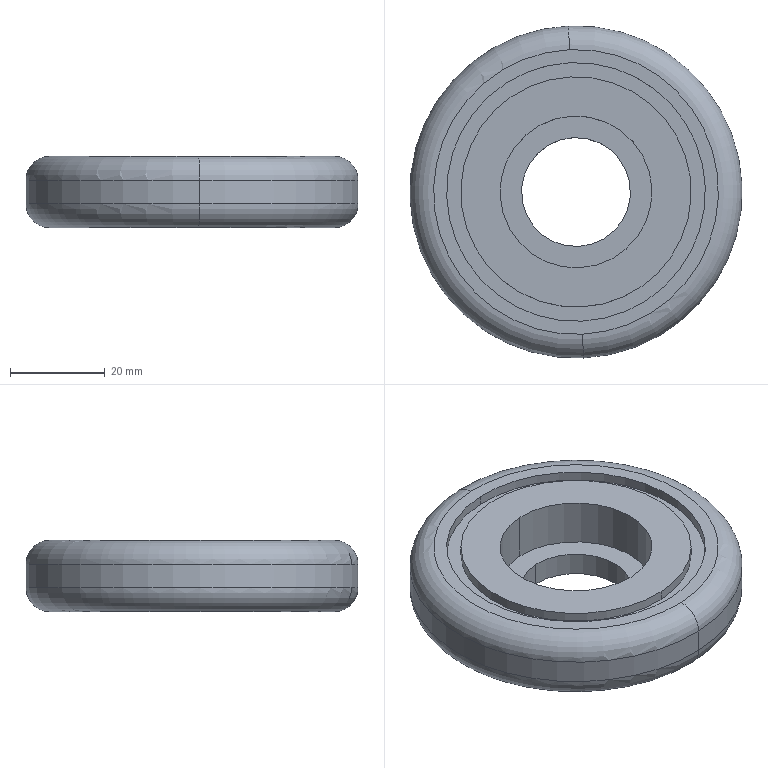Component | SolidWorks | RearWheel-1 | 1 solid | 25 faces | box 70 x 70 x 15 mm | volume 43388 mm3 | cylinder 14 | plane 7 | torus 4 | commonest cylinder face diameters 48.501 x4 54.501 x4 22.942 x2 32.008 x2 70 x2
STEP:
#1=COLOUR_RGB('',0.7922,0.8196,0.9333);
#2=FILL_AREA_STYLE_COLOUR('',#1);
#3=FILL_AREA_STYLE('',(#2));
#4=SURFACE_STYLE_FILL_AREA(#3);
#5=SURFACE_SIDE_STYLE('',(#4));
#6=SURFACE_STYLE_USAGE(.BOTH.,#5);
#7=PRESENTATION_STYLE_ASSIGNMENT((#6));
#8=CARTESIAN_POINT('',(7.614,-0.9245,-0.05906));
#9=VERTEX_POINT('',#8);
#10=CARTESIAN_POINT('',(7.573,-0.02218,-0.05906));
#11=VERTEX_POINT('',#10);
#12=CARTESIAN_POINT('',(7.594,-0.4733,-0.05906));
#13=DIRECTION('',(0.,0.,1.));
#14=DIRECTION('',(-0.04542,0.999,0.));
#15=AXIS2_PLACEMENT_3D('',#12,#13,#14);
#16=CIRCLE('',#15,0.4516);
#17=EDGE_CURVE('',#9,#11,#16,.T.);
#18=ORIENTED_EDGE('',*,*,#17,.T.);
#19=CARTESIAN_POINT('',(7.573,-0.02218,-0.2559));
#20=VERTEX_POINT('',#19);
#21=CARTESIAN_POINT('',(7.573,-0.02218,0.1378));
#22=DIRECTION('',(0.,0.,-1.));
#23=VECTOR('',#22,39.37);
#24=LINE('',#21,#23);
#25=EDGE_CURVE('',#11,#20,#24,.T.);
#26=ORIENTED_EDGE('',*,*,#25,.T.);
#27=CARTESIAN_POINT('',(7.614,-0.9245,-0.2559));
#28=VERTEX_POINT('',#27);
#29=CARTESIAN_POINT('',(7.594,-0.4733,-0.2559));
#30=DIRECTION('',(0.,0.,-1.));
#31=DIRECTION('',(0.04542,-0.999,0.));
#32=AXIS2_PLACEMENT_3D('',#29,#30,#31);
#33=CIRCLE('',#32,0.4516);
#34=EDGE_CURVE('',#20,#28,#33,.T.);
#35=ORIENTED_EDGE('',*,*,#34,.T.);
#36=CARTESIAN_POINT('',(7.614,-0.9245,0.1378));
#37=DIRECTION('',(0.,0.,-1.));
#38=VECTOR('',#37,39.37);
#39=LINE('',#36,#38);
#40=EDGE_CURVE('',#9,#28,#39,.T.);
#41=ORIENTED_EDGE('',*,*,#40,.F.);
#42=EDGE_LOOP('',(#18,#26,#35,#41));
#43=FACE_OUTER_BOUND('',#42,.T.);
#44=CARTESIAN_POINT('',(7.594,-0.4733,0.1378));
#45=DIRECTION('',(0.,0.,-1.));
#46=DIRECTION('',(0.04542,-0.999,0.));
#47=AXIS2_PLACEMENT_3D('',#44,#45,#46);
#48=CYLINDRICAL_SURFACE('',#47,0.4516);
#49=ADVANCED_FACE('',(#43),#48,.F.);
#50=CARTESIAN_POINT('',(7.622,-1.103,-0.05906));
#51=VERTEX_POINT('',#50);
#52=CARTESIAN_POINT('',(7.565,0.1561,-0.05906));
#53=VERTEX_POINT('',#52);
#54=CARTESIAN_POINT('',(7.594,-0.4733,-0.05906));
#55=DIRECTION('',(0.,0.,1.));
#56=DIRECTION('',(-0.04542,0.999,0.));
#57=AXIS2_PLACEMENT_3D('',#54,#55,#56);
#58=CIRCLE('',#57,0.6301);
#59=EDGE_CURVE('',#51,#53,#58,.T.);
#60=ORIENTED_EDGE('',*,*,#59,.F.);
#61=CARTESIAN_POINT('',(7.622,-1.103,0.3346));
#62=VERTEX_POINT('',#61);
#63=CARTESIAN_POINT('',(7.622,-1.103,-0.05906));
#64=DIRECTION('',(0.,0.,1.));
#65=VECTOR('',#64,39.37);
#66=LINE('',#63,#65);
#67=EDGE_CURVE('',#51,#62,#66,.T.);
#68=ORIENTED_EDGE('',*,*,#67,.T.);
#69=CARTESIAN_POINT('',(7.565,0.1561,0.3346));
#70=VERTEX_POINT('',#69);
#71=CARTESIAN_POINT('',(7.594,-0.4733,0.3346));
#72=DIRECTION('',(0.,0.,1.));
#73=DIRECTION('',(-0.04542,0.999,0.));
#74=AXIS2_PLACEMENT_3D('',#71,#72,#73);
#75=CIRCLE('',#74,0.6301);
#76=EDGE_CURVE('',#62,#70,#75,.T.);
#77=ORIENTED_EDGE('',*,*,#76,.T.);
#78=CARTESIAN_POINT('',(7.565,0.1561,-0.05906));
#79=DIRECTION('',(0.,0.,1.));
#80=VECTOR('',#79,39.37);
#81=LINE('',#78,#80);
#82=EDGE_CURVE('',#53,#70,#81,.T.);
#83=ORIENTED_EDGE('',*,*,#82,.F.);
#84=EDGE_LOOP('',(#60,#68,#77,#83));
#85=FACE_OUTER_BOUND('',#84,.T.);
#86=CARTESIAN_POINT('',(7.594,-0.4733,-0.05906));
#87=DIRECTION('',(0.,0.,1.));
#88=DIRECTION('',(-0.04542,0.999,0.));
#89=AXIS2_PLACEMENT_3D('',#86,#87,#88);
#90=CYLINDRICAL_SURFACE('',#89,0.6301);
#91=ADVANCED_FACE('',(#85),#90,.F.);
#92=CARTESIAN_POINT('',(7.637,-1.427,0.2559));
#93=VERTEX_POINT('',#92);
#94=CARTESIAN_POINT('',(7.55,0.4804,0.2559));
#95=VERTEX_POINT('',#94);
#96=CARTESIAN_POINT('',(7.594,-0.4733,0.2559));
#97=DIRECTION('',(0.,0.,-1.));
#98=DIRECTION('',(0.04542,-0.999,0.));
#99=AXIS2_PLACEMENT_3D('',#96,#97,#98);
#100=CIRCLE('',#99,0.9548);
#101=EDGE_CURVE('',#93,#95,#100,.T.);
#102=ORIENTED_EDGE('',*,*,#101,.F.);
#103=CARTESIAN_POINT('',(7.637,-1.427,0.3346));
#104=VERTEX_POINT('',#103);
#105=CARTESIAN_POINT('',(7.637,-1.427,0.2559));
#106=DIRECTION('',(0.,0.,1.));
#107=VECTOR('',#106,39.37);
#108=LINE('',#105,#107);
#109=EDGE_CURVE('',#93,#104,#108,.T.);
#110=ORIENTED_EDGE('',*,*,#109,.T.);
#111=CARTESIAN_POINT('',(7.55,0.4804,0.3346));
#112=VERTEX_POINT('',#111);
#113=CARTESIAN_POINT('',(7.594,-0.4733,0.3346));
#114=DIRECTION('',(0.,0.,-1.));
#115=DIRECTION('',(0.04542,-0.999,0.));
#116=AXIS2_PLACEMENT_3D('',#113,#114,#115);
#117=CIRCLE('',#116,0.9548);
#118=EDGE_CURVE('',#104,#112,#117,.T.);
#119=ORIENTED_EDGE('',*,*,#118,.T.);
#120=CARTESIAN_POINT('',(7.55,0.4804,0.2559));
#121=DIRECTION('',(0.,0.,1.));
#122=VECTOR('',#121,39.37);
#123=LINE('',#120,#122);
#124=EDGE_CURVE('',#95,#112,#123,.T.);
#125=ORIENTED_EDGE('',*,*,#124,.F.);
#126=EDGE_LOOP('',(#102,#110,#119,#125));
#127=FACE_OUTER_BOUND('',#126,.T.);
#128=CARTESIAN_POINT('',(7.594,-0.4733,0.2559));
#129=DIRECTION('',(0.,0.,1.));
#130=DIRECTION('',(-0.04542,0.999,0.));
#131=AXIS2_PLACEMENT_3D('',#128,#129,#130);
#132=CYLINDRICAL_SURFACE('',#131,0.9548);
#133=ADVANCED_FACE('',(#127),#132,.T.);
#134=CARTESIAN_POINT('',(7.545,0.5984,0.2559));
#135=VERTEX_POINT('',#134);
#136=CARTESIAN_POINT('',(7.642,-1.545,0.2559));
#137=VERTEX_POINT('',#136);
#138=CARTESIAN_POINT('',(7.594,-0.4733,0.2559));
#139=DIRECTION('',(0.,0.,-1.));
#140=DIRECTION('',(0.04542,-0.999,0.));
#141=AXIS2_PLACEMENT_3D('',#138,#139,#140);
#142=CIRCLE('',#141,1.073);
#143=EDGE_CURVE('',#135,#137,#142,.T.);
#144=ORIENTED_EDGE('',*,*,#143,.T.);
#145=CARTESIAN_POINT('',(7.642,-1.545,0.3346));
#146=VERTEX_POINT('',#145);
#147=CARTESIAN_POINT('',(7.642,-1.545,0.2559));
#148=DIRECTION('',(0.,0.,1.));
#149=VECTOR('',#148,39.37);
#150=LINE('',#147,#149);
#151=EDGE_CURVE('',#137,#146,#150,.T.);
#152=ORIENTED_EDGE('',*,*,#151,.T.);
#153=CARTESIAN_POINT('',(7.545,0.5984,0.3346));
#154=VERTEX_POINT('',#153);
#155=CARTESIAN_POINT('',(7.594,-0.4733,0.3346));
#156=DIRECTION('',(0.,0.,-1.));
#157=DIRECTION('',(0.04542,-0.999,0.));
#158=AXIS2_PLACEMENT_3D('',#155,#156,#157);
#159=CIRCLE('',#158,1.073);
#160=EDGE_CURVE('',#154,#146,#159,.T.);
#161=ORIENTED_EDGE('',*,*,#160,.F.);
#162=CARTESIAN_POINT('',(7.545,0.5984,0.2559));
#163=DIRECTION('',(0.,0.,1.));
#164=VECTOR('',#163,39.37);
#165=LINE('',#162,#164);
#166=EDGE_CURVE('',#135,#154,#165,.T.);
#167=ORIENTED_EDGE('',*,*,#166,.F.);
#168=EDGE_LOOP('',(#144,#152,#161,#167));
#169=FACE_OUTER_BOUND('',#168,.T.);
#170=CARTESIAN_POINT('',(7.594,-0.4733,0.2559));
#171=DIRECTION('',(0.,0.,1.));
#172=DIRECTION('',(-0.04542,0.999,0.));
#173=AXIS2_PLACEMENT_3D('',#170,#171,#172);
#174=CYLINDRICAL_SURFACE('',#173,1.073);
#175=ADVANCED_FACE('',(#169),#174,.F.);
#176=CARTESIAN_POINT('',(7.637,-1.427,-0.1772));
#177=VERTEX_POINT('',#176);
#178=CARTESIAN_POINT('',(7.55,0.4804,-0.1772));
#179=VERTEX_POINT('',#178);
#180=CARTESIAN_POINT('',(7.594,-0.4733,-0.1772));
#181=DIRECTION('',(0.,0.,-1.));
#182=DIRECTION('',(0.04542,-0.999,0.));
#183=AXIS2_PLACEMENT_3D('',#180,#181,#182);
#184=CIRCLE('',#183,0.9548);
#185=EDGE_CURVE('',#177,#179,#184,.T.);
#186=ORIENTED_EDGE('',*,*,#185,.T.);
#187=CARTESIAN_POINT('',(7.55,0.4804,-0.2559));
#188=VERTEX_POINT('',#187);
#189=CARTESIAN_POINT('',(7.55,0.4804,-0.1772));
#190=DIRECTION('',(0.,0.,-1.));
#191=VECTOR('',#190,39.37);
#192=LINE('',#189,#191);
#193=EDGE_CURVE('',#179,#188,#192,.T.);
#194=ORIENTED_EDGE('',*,*,#193,.T.);
#195=CARTESIAN_POINT('',(7.637,-1.427,-0.2559));
#196=VERTEX_POINT('',#195);
#197=CARTESIAN_POINT('',(7.594,-0.4733,-0.2559));
#198=DIRECTION('',(0.,0.,-1.));
#199=DIRECTION('',(0.04542,-0.999,0.));
#200=AXIS2_PLACEMENT_3D('',#197,#198,#199);
#201=CIRCLE('',#200,0.9548);
#202=EDGE_CURVE('',#196,#188,#201,.T.);
#203=ORIENTED_EDGE('',*,*,#202,.F.);
#204=CARTESIAN_POINT('',(7.637,-1.427,-0.1772));
#205=DIRECTION('',(0.,0.,-1.));
#206=VECTOR('',#205,39.37);
#207=LINE('',#204,#206);
#208=EDGE_CURVE('',#177,#196,#207,.T.);
#209=ORIENTED_EDGE('',*,*,#208,.F.);
#210=EDGE_LOOP('',(#186,#194,#203,#209));
#211=FACE_OUTER_BOUND('',#210,.T.);
#212=CARTESIAN_POINT('',(7.594,-0.4733,-0.1772));
#213=DIRECTION('',(0.,0.,-1.));
#214=DIRECTION('',(0.04542,-0.999,0.));
#215=AXIS2_PLACEMENT_3D('',#212,#213,#214);
#216=CYLINDRICAL_SURFACE('',#215,0.9548);
#217=ADVANCED_FACE('',(#211),#216,.T.);
#218=CARTESIAN_POINT('',(7.545,0.5984,-0.1772));
#219=VERTEX_POINT('',#218);
#220=CARTESIAN_POINT('',(7.642,-1.545,-0.1772));
#221=VERTEX_POINT('',#220);
#222=CARTESIAN_POINT('',(7.594,-0.4733,-0.1772));
#223=DIRECTION('',(0.,0.,-1.));
#224=DIRECTION('',(0.04542,-0.999,0.));
#225=AXIS2_PLACEMENT_3D('',#222,#223,#224);
#226=CIRCLE('',#225,1.073);
#227=EDGE_CURVE('',#219,#221,#226,.T.);
#228=ORIENTED_EDGE('',*,*,#227,.F.);
#229=CARTESIAN_POINT('',(7.545,0.5984,-0.2559));
#230=VERTEX_POINT('',#229);
#231=CARTESIAN_POINT('',(7.545,0.5984,-0.1772));
#232=DIRECTION('',(0.,0.,-1.));
#233=VECTOR('',#232,39.37);
#234=LINE('',#231,#233);
#235=EDGE_CURVE('',#219,#230,#234,.T.);
#236=ORIENTED_EDGE('',*,*,#235,.T.);
#237=CARTESIAN_POINT('',(7.642,-1.545,-0.2559));
#238=VERTEX_POINT('',#237);
#239=CARTESIAN_POINT('',(7.594,-0.4733,-0.2559));
#240=DIRECTION('',(0.,0.,-1.));
#241=DIRECTION('',(0.04542,-0.999,0.));
#242=AXIS2_PLACEMENT_3D('',#239,#240,#241);
#243=CIRCLE('',#242,1.073);
#244=EDGE_CURVE('',#230,#238,#243,.T.);
#245=ORIENTED_EDGE('',*,*,#244,.T.);
#246=CARTESIAN_POINT('',(7.642,-1.545,-0.1772));
#247=DIRECTION('',(0.,0.,-1.));
#248=VECTOR('',#247,39.37);
#249=LINE('',#246,#248);
#250=EDGE_CURVE('',#221,#238,#249,.T.);
#251=ORIENTED_EDGE('',*,*,#250,.F.);
#252=EDGE_LOOP('',(#228,#236,#245,#251));
#253=FACE_OUTER_BOUND('',#252,.T.);
#254=CARTESIAN_POINT('',(7.594,-0.4733,-0.1772));
#255=DIRECTION('',(0.,0.,-1.));
#256=DIRECTION('',(0.04542,-0.999,0.));
#257=AXIS2_PLACEMENT_3D('',#254,#255,#256);
#258=CYLINDRICAL_SURFACE('',#257,1.073);
#259=ADVANCED_FACE('',(#253),#258,.F.);
#260=CARTESIAN_POINT('',(7.656,-1.85,0.1378));
#261=VERTEX_POINT('',#260);
#262=CARTESIAN_POINT('',(7.531,0.9032,0.1378));
#263=VERTEX_POINT('',#262);
#264=CARTESIAN_POINT('',(7.594,-0.4733,0.1378));
#265=DIRECTION('',(0.,0.,-1.));
#266=DIRECTION('',(-0.04542,0.999,0.));
#267=AXIS2_PLACEMENT_3D('',#264,#265,#266);
#268=CIRCLE('',#267,1.378);
#269=EDGE_CURVE('',#261,#263,#268,.T.);
#270=ORIENTED_EDGE('',*,*,#269,.F.);
#271=CARTESIAN_POINT('',(7.647,-1.653,0.3346));
#272=VERTEX_POINT('',#271);
#273=CARTESIAN_POINT('',(7.647,-1.653,0.1378));
#274=DIRECTION('',(-0.999,-0.04542,0.));
#275=DIRECTION('',(0.04542,-0.999,0.));
#276=AXIS2_PLACEMENT_3D('',#273,#274,#275);
#277=CIRCLE('',#276,0.1969);
#278=EDGE_CURVE('',#261,#272,#277,.T.);
#279=ORIENTED_EDGE('',*,*,#278,.T.);
#280=CARTESIAN_POINT('',(7.54,0.7066,0.3346));
#281=VERTEX_POINT('',#280);
#282=CARTESIAN_POINT('',(7.594,-0.4733,0.3346));
#283=DIRECTION('',(0.,0.,1.));
#284=DIRECTION('',(-0.04542,0.999,0.));
#285=AXIS2_PLACEMENT_3D('',#282,#283,#284);
#286=CIRCLE('',#285,1.181);
#287=EDGE_CURVE('',#281,#272,#286,.T.);
#288=ORIENTED_EDGE('',*,*,#287,.F.);
#289=CARTESIAN_POINT('',(7.54,0.7066,0.1378));
#290=DIRECTION('',(0.999,0.04542,0.));
#291=DIRECTION('',(-0.04542,0.999,0.));
#292=AXIS2_PLACEMENT_3D('',#289,#290,#291);
#293=CIRCLE('',#292,0.1969);
#294=EDGE_CURVE('',#263,#281,#293,.T.);
#295=ORIENTED_EDGE('',*,*,#294,.F.);
#296=EDGE_LOOP('',(#270,#279,#288,#295));
#297=FACE_OUTER_BOUND('',#296,.T.);
#298=CARTESIAN_POINT('',(7.594,-0.4733,0.1378));
#299=DIRECTION('',(0.,0.,1.));
#300=DIRECTION('',(-0.04542,0.999,0.));
#301=AXIS2_PLACEMENT_3D('',#298,#299,#300);
#302=TOROIDAL_SURFACE('',#301,1.181,0.1969);
#303=ADVANCED_FACE('',(#297),#302,.T.);
#304=CARTESIAN_POINT('',(7.54,0.7066,-0.2559));
#305=VERTEX_POINT('',#304);
#306=CARTESIAN_POINT('',(7.647,-1.653,-0.2559));
#307=VERTEX_POINT('',#306);
#308=CARTESIAN_POINT('',(7.594,-0.4733,-0.2559));
#309=DIRECTION('',(0.,0.,1.));
#310=DIRECTION('',(-0.04542,0.999,0.));
#311=AXIS2_PLACEMENT_3D('',#308,#309,#310);
#312=CIRCLE('',#311,1.181);
#313=EDGE_CURVE('',#305,#307,#312,.T.);
#314=ORIENTED_EDGE('',*,*,#313,.T.);
#315=CARTESIAN_POINT('',(7.656,-1.85,-0.05906));
#316=VERTEX_POINT('',#315);
#317=CARTESIAN_POINT('',(7.647,-1.653,-0.05906));
#318=DIRECTION('',(-0.999,-0.04542,0.));
#319=DIRECTION('',(0.04542,-0.999,0.));
#320=AXIS2_PLACEMENT_3D('',#317,#318,#319);
#321=CIRCLE('',#320,0.1969);
#322=EDGE_CURVE('',#307,#316,#321,.T.);
#323=ORIENTED_EDGE('',*,*,#322,.T.);
#324=CARTESIAN_POINT('',(7.531,0.9032,-0.05906));
#325=VERTEX_POINT('',#324);
#326=CARTESIAN_POINT('',(7.594,-0.4733,-0.05906));
#327=DIRECTION('',(0.,0.,1.));
#328=DIRECTION('',(-0.04542,0.999,0.));
#329=AXIS2_PLACEMENT_3D('',#326,#327,#328);
#330=CIRCLE('',#329,1.378);
#331=EDGE_CURVE('',#325,#316,#330,.T.);
#332=ORIENTED_EDGE('',*,*,#331,.F.);
#333=CARTESIAN_POINT('',(7.54,0.7066,-0.05906));
#334=DIRECTION('',(0.999,0.04542,0.));
#335=DIRECTION('',(-0.04542,0.999,0.));
#336=AXIS2_PLACEMENT_3D('',#333,#334,#335);
#337=CIRCLE('',#336,0.1969);
#338=EDGE_CURVE('',#305,#325,#337,.T.);
#339=ORIENTED_EDGE('',*,*,#338,.F.);
#340=EDGE_LOOP('',(#314,#323,#332,#339));
#341=FACE_OUTER_BOUND('',#340,.T.);
#342=CARTESIAN_POINT('',(7.594,-0.4733,-0.05906));
#343=DIRECTION('',(0.,0.,1.));
#344=DIRECTION('',(-0.04542,0.999,0.));
#345=AXIS2_PLACEMENT_3D('',#342,#343,#344);
#346=TOROIDAL_SURFACE('',#345,1.181,0.1969);
#347=ADVANCED_FACE('',(#341),#346,.T.);
#348=ORIENTED_EDGE('',*,*,#269,.T.);
#349=CARTESIAN_POINT('',(7.531,0.9032,0.3346));
#350=DIRECTION('',(0.,0.,-1.));
#351=VECTOR('',#350,39.37);
#352=LINE('',#349,#351);
#353=EDGE_CURVE('',#263,#325,#352,.T.);
#354=ORIENTED_EDGE('',*,*,#353,.T.);
#355=ORIENTED_EDGE('',*,*,#331,.T.);
#356=CARTESIAN_POINT('',(7.656,-1.85,0.3346));
#357=DIRECTION('',(0.,0.,-1.));
#358=VECTOR('',#357,39.37);
#359=LINE('',#356,#358);
#360=EDGE_CURVE('',#261,#316,#359,.T.);
#361=ORIENTED_EDGE('',*,*,#360,.F.);
#362=EDGE_LOOP('',(#348,#354,#355,#361));
#363=FACE_OUTER_BOUND('',#362,.T.);
#364=CARTESIAN_POINT('',(7.594,-0.4733,0.3346));
#365=DIRECTION('',(0.,0.,-1.));
#366=DIRECTION('',(0.04542,-0.999,0.));
#367=AXIS2_PLACEMENT_3D('',#364,#365,#366);
#368=CYLINDRICAL_SURFACE('',#367,1.378);
#369=ADVANCED_FACE('',(#363),#368,.T.);
#370=CARTESIAN_POINT('',(7.594,-0.4733,0.3346));
#371=DIRECTION('',(0.,0.,1.));
#372=DIRECTION('',(-0.04542,0.999,0.));
#373=AXIS2_PLACEMENT_3D('',#370,#371,#372);
#374=CIRCLE('',#373,0.6301);
#375=EDGE_CURVE('',#70,#62,#374,.T.);
#376=ORIENTED_EDGE('',*,*,#375,.F.);
#377=ORIENTED_EDGE('',*,*,#76,.F.);
#378=EDGE_LOOP('',(#376,#377));
#379=FACE_BOUND('',#378,.T.);
#380=CARTESIAN_POINT('',(7.594,-0.4733,0.3346));
#381=DIRECTION('',(0.,0.,-1.));
#382=DIRECTION('',(0.04542,-0.999,0.));
#383=AXIS2_PLACEMENT_3D('',#380,#381,#382);
#384=CIRCLE('',#383,0.9548);
#385=EDGE_CURVE('',#112,#104,#384,.T.);
#386=ORIENTED_EDGE('',*,*,#385,.F.);
#387=ORIENTED_EDGE('',*,*,#118,.F.);
#388=EDGE_LOOP('',(#386,#387));
#389=FACE_OUTER_BOUND('',#388,.T.);
#390=CARTESIAN_POINT('',(7.594,-0.4733,0.3346));
#391=DIRECTION('',(0.,0.,1.));
#392=DIRECTION('',(-0.04542,0.999,0.));
#393=AXIS2_PLACEMENT_3D('',#390,#391,#392);
#394=PLANE('',#393);
#395=ADVANCED_FACE('',(#379,#389),#394,.T.);
#396=CARTESIAN_POINT('',(7.594,-0.4733,-0.2559));
#397=DIRECTION('',(0.,0.,-1.));
#398=DIRECTION('',(0.04542,-0.999,0.));
#399=AXIS2_PLACEMENT_3D('',#396,#397,#398);
#400=CIRCLE('',#399,0.4516);
#401=EDGE_CURVE('',#28,#20,#400,.T.);
#402=ORIENTED_EDGE('',*,*,#401,.F.);
#403=ORIENTED_EDGE('',*,*,#34,.F.);
#404=EDGE_LOOP('',(#402,#403));
#405=FACE_BOUND('',#404,.T.);
#406=ORIENTED_EDGE('',*,*,#202,.T.);
#407=CARTESIAN_POINT('',(7.594,-0.4733,-0.2559));
#408=DIRECTION('',(0.,0.,-1.));
#409=DIRECTION('',(0.04542,-0.999,0.));
#410=AXIS2_PLACEMENT_3D('',#407,#408,#409);
#411=CIRCLE('',#410,0.9548);
#412=EDGE_CURVE('',#188,#196,#411,.T.);
#413=ORIENTED_EDGE('',*,*,#412,.T.);
#414=EDGE_LOOP('',(#406,#413));
#415=FACE_OUTER_BOUND('',#414,.T.);
#416=CARTESIAN_POINT('',(7.594,-0.4733,-0.2559));
#417=DIRECTION('',(0.,0.,1.));
#418=DIRECTION('',(-0.04542,0.999,0.));
#419=AXIS2_PLACEMENT_3D('',#416,#417,#418);
#420=PLANE('',#419);
#421=ADVANCED_FACE('',(#405,#415),#420,.F.);
#422=ORIENTED_EDGE('',*,*,#353,.F.);
#423=CARTESIAN_POINT('',(7.594,-0.4733,0.1378));
#424=DIRECTION('',(0.,0.,-1.));
#425=DIRECTION('',(-0.04542,0.999,0.));
#426=AXIS2_PLACEMENT_3D('',#423,#424,#425);
#427=CIRCLE('',#426,1.378);
#428=EDGE_CURVE('',#263,#261,#427,.T.);
#429=ORIENTED_EDGE('',*,*,#428,.T.);
#430=ORIENTED_EDGE('',*,*,#360,.T.);
#431=CARTESIAN_POINT('',(7.594,-0.4733,-0.05906));
#432=DIRECTION('',(0.,0.,1.));
#433=DIRECTION('',(-0.04542,0.999,0.));
#434=AXIS2_PLACEMENT_3D('',#431,#432,#433);
#435=CIRCLE('',#434,1.378);
#436=EDGE_CURVE('',#316,#325,#435,.T.);
#437=ORIENTED_EDGE('',*,*,#436,.T.);
#438=EDGE_LOOP('',(#422,#429,#430,#437));
#439=FACE_OUTER_BOUND('',#438,.T.);
#440=CARTESIAN_POINT('',(7.594,-0.4733,0.3346));
#441=DIRECTION('',(0.,0.,-1.));
#442=DIRECTION('',(0.04542,-0.999,0.));
#443=AXIS2_PLACEMENT_3D('',#440,#441,#442);
#444=CYLINDRICAL_SURFACE('',#443,1.378);
#445=ADVANCED_FACE('',(#439),#444,.T.);
#446=ORIENTED_EDGE('',*,*,#322,.F.);
#447=CARTESIAN_POINT('',(7.594,-0.4733,-0.2559));
#448=DIRECTION('',(0.,0.,1.));
#449=DIRECTION('',(-0.04542,0.999,0.));
#450=AXIS2_PLACEMENT_3D('',#447,#448,#449);
#451=CIRCLE('',#450,1.181);
#452=EDGE_CURVE('',#307,#305,#451,.T.);
#453=ORIENTED_EDGE('',*,*,#452,.T.);
#454=ORIENTED_EDGE('',*,*,#338,.T.);
#455=ORIENTED_EDGE('',*,*,#436,.F.);
#456=EDGE_LOOP('',(#446,#453,#454,#455));
#457=FACE_OUTER_BOUND('',#456,.T.);
#458=CARTESIAN_POINT('',(7.594,-0.4733,-0.05906));
#459=DIRECTION('',(0.,0.,1.));
#460=DIRECTION('',(-0.04542,0.999,0.));
#461=AXIS2_PLACEMENT_3D('',#458,#459,#460);
#462=TOROIDAL_SURFACE('',#461,1.181,0.1969);
#463=ADVANCED_FACE('',(#457),#462,.T.);
#464=ORIENTED_EDGE('',*,*,#278,.F.);
#465=ORIENTED_EDGE('',*,*,#428,.F.);
#466=ORIENTED_EDGE('',*,*,#294,.T.);
#467=CARTESIAN_POINT('',(7.594,-0.4733,0.3346));
#468=DIRECTION('',(0.,0.,1.));
#469=DIRECTION('',(-0.04542,0.999,0.));
#470=AXIS2_PLACEMENT_3D('',#467,#468,#469);
#471=CIRCLE('',#470,1.181);
#472=EDGE_CURVE('',#272,#281,#471,.T.);
#473=ORIENTED_EDGE('',*,*,#472,.F.);
#474=EDGE_LOOP('',(#464,#465,#466,#473));
#475=FACE_OUTER_BOUND('',#474,.T.);
#476=CARTESIAN_POINT('',(7.594,-0.4733,0.1378));
#477=DIRECTION('',(0.,0.,1.));
#478=DIRECTION('',(-0.04542,0.999,0.));
#479=AXIS2_PLACEMENT_3D('',#476,#477,#478);
#480=TOROIDAL_SURFACE('',#479,1.181,0.1969);
#481=ADVANCED_FACE('',(#475),#480,.T.);
#482=ORIENTED_EDGE('',*,*,#160,.T.);
#483=CARTESIAN_POINT('',(7.594,-0.4733,0.3346));
#484=DIRECTION('',(0.,0.,-1.));
#485=DIRECTION('',(0.04542,-0.999,0.));
#486=AXIS2_PLACEMENT_3D('',#483,#484,#485);
#487=CIRCLE('',#486,1.073);
#488=EDGE_CURVE('',#146,#154,#487,.T.);
#489=ORIENTED_EDGE('',*,*,#488,.T.);
#490=EDGE_LOOP('',(#482,#489));
#491=FACE_BOUND('',#490,.T.);
#492=ORIENTED_EDGE('',*,*,#287,.T.);
#493=ORIENTED_EDGE('',*,*,#472,.T.);
#494=EDGE_LOOP('',(#492,#493));
#495=FACE_OUTER_BOUND('',#494,.T.);
#496=CARTESIAN_POINT('',(7.594,-0.4733,0.3346));
#497=DIRECTION('',(0.,0.,1.));
#498=DIRECTION('',(-0.04542,0.999,0.));
#499=AXIS2_PLACEMENT_3D('',#496,#497,#498);
#500=PLANE('',#499);
#501=ADVANCED_FACE('',(#491,#495),#500,.T.);
#502=CARTESIAN_POINT('',(7.594,-0.4733,-0.2559));
#503=DIRECTION('',(0.,0.,-1.));
#504=DIRECTION('',(0.04542,-0.999,0.));
#505=AXIS2_PLACEMENT_3D('',#502,#503,#504);
#506=CIRCLE('',#505,1.073);
#507=EDGE_CURVE('',#238,#230,#506,.T.);
#508=ORIENTED_EDGE('',*,*,#507,.F.);
#509=ORIENTED_EDGE('',*,*,#244,.F.);
#510=EDGE_LOOP('',(#508,#509));
#511=FACE_BOUND('',#510,.T.);
#512=ORIENTED_EDGE('',*,*,#313,.F.);
#513=ORIENTED_EDGE('',*,*,#452,.F.);
#514=EDGE_LOOP('',(#512,#513));
#515=FACE_OUTER_BOUND('',#514,.T.);
#516=CARTESIAN_POINT('',(7.594,-0.4733,-0.2559));
#517=DIRECTION('',(0.,0.,1.));
#518=DIRECTION('',(-0.04542,0.999,0.));
#519=AXIS2_PLACEMENT_3D('',#516,#517,#518);
#520=PLANE('',#519);
#521=ADVANCED_FACE('',(#511,#515),#520,.F.);
#522=ORIENTED_EDGE('',*,*,#235,.F.);
#523=CARTESIAN_POINT('',(7.594,-0.4733,-0.1772));
#524=DIRECTION('',(0.,0.,-1.));
#525=DIRECTION('',(0.04542,-0.999,0.));
#526=AXIS2_PLACEMENT_3D('',#523,#524,#525);
#527=CIRCLE('',#526,1.073);
#528=EDGE_CURVE('',#221,#219,#527,.T.);
#529=ORIENTED_EDGE('',*,*,#528,.F.);
#530=ORIENTED_EDGE('',*,*,#250,.T.);
#531=ORIENTED_EDGE('',*,*,#507,.T.);
#532=EDGE_LOOP('',(#522,#529,#530,#531));
#533=FACE_OUTER_BOUND('',#532,.T.);
#534=CARTESIAN_POINT('',(7.594,-0.4733,-0.1772));
#535=DIRECTION('',(0.,0.,-1.));
#536=DIRECTION('',(0.04542,-0.999,0.));
#537=AXIS2_PLACEMENT_3D('',#534,#535,#536);
#538=CYLINDRICAL_SURFACE('',#537,1.073);
#539=ADVANCED_FACE('',(#533),#538,.F.);
#540=ORIENTED_EDGE('',*,*,#185,.F.);
#541=CARTESIAN_POINT('',(7.594,-0.4733,-0.1772));
#542=DIRECTION('',(0.,0.,-1.));
#543=DIRECTION('',(0.04542,-0.999,0.));
#544=AXIS2_PLACEMENT_3D('',#541,#542,#543);
#545=CIRCLE('',#544,0.9548);
#546=EDGE_CURVE('',#179,#177,#545,.T.);
#547=ORIENTED_EDGE('',*,*,#546,.F.);
#548=EDGE_LOOP('',(#540,#547));
#549=FACE_BOUND('',#548,.T.);
#550=ORIENTED_EDGE('',*,*,#528,.T.);
#551=ORIENTED_EDGE('',*,*,#227,.T.);
#552=EDGE_LOOP('',(#550,#551));
#553=FACE_OUTER_BOUND('',#552,.T.);
#554=CARTESIAN_POINT('',(7.594,-0.4733,-0.1772));
#555=DIRECTION('',(0.,0.,-1.));
#556=DIRECTION('',(0.04542,-0.999,0.));
#557=AXIS2_PLACEMENT_3D('',#554,#555,#556);
#558=PLANE('',#557);
#559=ADVANCED_FACE('',(#549,#553),#558,.T.);
#560=ORIENTED_EDGE('',*,*,#193,.F.);
#561=ORIENTED_EDGE('',*,*,#546,.T.);
#562=ORIENTED_EDGE('',*,*,#208,.T.);
#563=ORIENTED_EDGE('',*,*,#412,.F.);
#564=EDGE_LOOP('',(#560,#561,#562,#563));
#565=FACE_OUTER_BOUND('',#564,.T.);
#566=CARTESIAN_POINT('',(7.594,-0.4733,-0.1772));
#567=DIRECTION('',(0.,0.,-1.));
#568=DIRECTION('',(0.04542,-0.999,0.));
#569=AXIS2_PLACEMENT_3D('',#566,#567,#568);
#570=CYLINDRICAL_SURFACE('',#569,0.9548);
#571=ADVANCED_FACE('',(#565),#570,.T.);
#572=ORIENTED_EDGE('',*,*,#143,.F.);
#573=CARTESIAN_POINT('',(7.594,-0.4733,0.2559));
#574=DIRECTION('',(0.,0.,-1.));
#575=DIRECTION('',(0.04542,-0.999,0.));
#576=AXIS2_PLACEMENT_3D('',#573,#574,#575);
#577=CIRCLE('',#576,1.073);
#578=EDGE_CURVE('',#137,#135,#577,.T.);
#579=ORIENTED_EDGE('',*,*,#578,.F.);
#580=EDGE_LOOP('',(#572,#579));
#581=FACE_OUTER_BOUND('',#580,.T.);
#582=CARTESIAN_POINT('',(7.594,-0.4733,0.2559));
#583=DIRECTION('',(0.,0.,-1.));
#584=DIRECTION('',(0.04542,-0.999,0.));
#585=AXIS2_PLACEMENT_3D('',#582,#583,#584);
#586=CIRCLE('',#585,0.9548);
#587=EDGE_CURVE('',#95,#93,#586,.T.);
#588=ORIENTED_EDGE('',*,*,#587,.T.);
#589=ORIENTED_EDGE('',*,*,#101,.T.);
#590=EDGE_LOOP('',(#588,#589));
#591=FACE_BOUND('',#590,.T.);
#592=CARTESIAN_POINT('',(7.594,-0.4733,0.2559));
#593=DIRECTION('',(0.,0.,-1.));
#594=DIRECTION('',(0.04542,-0.999,0.));
#595=AXIS2_PLACEMENT_3D('',#592,#593,#594);
#596=PLANE('',#595);
#597=ADVANCED_FACE('',(#581,#591),#596,.F.);
#598=ORIENTED_EDGE('',*,*,#151,.F.);
#599=ORIENTED_EDGE('',*,*,#578,.T.);
#600=ORIENTED_EDGE('',*,*,#166,.T.);
#601=ORIENTED_EDGE('',*,*,#488,.F.);
#602=EDGE_LOOP('',(#598,#599,#600,#601));
#603=FACE_OUTER_BOUND('',#602,.T.);
#604=CARTESIAN_POINT('',(7.594,-0.4733,0.2559));
#605=DIRECTION('',(0.,0.,1.));
#606=DIRECTION('',(-0.04542,0.999,0.));
#607=AXIS2_PLACEMENT_3D('',#604,#605,#606);
#608=CYLINDRICAL_SURFACE('',#607,1.073);
#609=ADVANCED_FACE('',(#603),#608,.F.);
#610=ORIENTED_EDGE('',*,*,#109,.F.);
#611=ORIENTED_EDGE('',*,*,#587,.F.);
#612=ORIENTED_EDGE('',*,*,#124,.T.);
#613=ORIENTED_EDGE('',*,*,#385,.T.);
#614=EDGE_LOOP('',(#610,#611,#612,#613));
#615=FACE_OUTER_BOUND('',#614,.T.);
#616=CARTESIAN_POINT('',(7.594,-0.4733,0.2559));
#617=DIRECTION('',(0.,0.,1.));
#618=DIRECTION('',(-0.04542,0.999,0.));
#619=AXIS2_PLACEMENT_3D('',#616,#617,#618);
#620=CYLINDRICAL_SURFACE('',#619,0.9548);
#621=ADVANCED_FACE('',(#615),#620,.T.);
#622=ORIENTED_EDGE('',*,*,#67,.F.);
#623=CARTESIAN_POINT('',(7.594,-0.4733,-0.05906));
#624=DIRECTION('',(0.,0.,1.));
#625=DIRECTION('',(-0.04542,0.999,0.));
#626=AXIS2_PLACEMENT_3D('',#623,#624,#625);
#627=CIRCLE('',#626,0.6301);
#628=EDGE_CURVE('',#53,#51,#627,.T.);
#629=ORIENTED_EDGE('',*,*,#628,.F.);
#630=ORIENTED_EDGE('',*,*,#82,.T.);
#631=ORIENTED_EDGE('',*,*,#375,.T.);
#632=EDGE_LOOP('',(#622,#629,#630,#631));
#633=FACE_OUTER_BOUND('',#632,.T.);
#634=CARTESIAN_POINT('',(7.594,-0.4733,-0.05906));
#635=DIRECTION('',(0.,0.,1.));
#636=DIRECTION('',(-0.04542,0.999,0.));
#637=AXIS2_PLACEMENT_3D('',#634,#635,#636);
#638=CYLINDRICAL_SURFACE('',#637,0.6301);
#639=ADVANCED_FACE('',(#633),#638,.F.);
#640=ORIENTED_EDGE('',*,*,#17,.F.);
#641=CARTESIAN_POINT('',(7.594,-0.4733,-0.05906));
#642=DIRECTION('',(0.,0.,1.));
#643=DIRECTION('',(-0.04542,0.999,0.));
#644=AXIS2_PLACEMENT_3D('',#641,#642,#643);
#645=CIRCLE('',#644,0.4516);
#646=EDGE_CURVE('',#11,#9,#645,.T.);
#647=ORIENTED_EDGE('',*,*,#646,.F.);
#648=EDGE_LOOP('',(#640,#647));
#649=FACE_BOUND('',#648,.T.);
#650=ORIENTED_EDGE('',*,*,#628,.T.);
#651=ORIENTED_EDGE('',*,*,#59,.T.);
#652=EDGE_LOOP('',(#650,#651));
#653=FACE_OUTER_BOUND('',#652,.T.);
#654=CARTESIAN_POINT('',(7.594,-0.4733,-0.05906));
#655=DIRECTION('',(0.,0.,1.));
#656=DIRECTION('',(-0.04542,0.999,0.));
#657=AXIS2_PLACEMENT_3D('',#654,#655,#656);
#658=PLANE('',#657);
#659=ADVANCED_FACE('',(#649,#653),#658,.T.);
#660=ORIENTED_EDGE('',*,*,#25,.F.);
#661=ORIENTED_EDGE('',*,*,#646,.T.);
#662=ORIENTED_EDGE('',*,*,#40,.T.);
#663=ORIENTED_EDGE('',*,*,#401,.T.);
#664=EDGE_LOOP('',(#660,#661,#662,#663));
#665=FACE_OUTER_BOUND('',#664,.T.);
#666=CARTESIAN_POINT('',(7.594,-0.4733,0.1378));
#667=DIRECTION('',(0.,0.,-1.));
#668=DIRECTION('',(0.04542,-0.999,0.));
#669=AXIS2_PLACEMENT_3D('',#666,#667,#668);
#670=CYLINDRICAL_SURFACE('',#669,0.4516);
#671=ADVANCED_FACE('',(#665),#670,.F.);
#672=CLOSED_SHELL('',(#49,#91,#133,#175,#217,#259,#303,#347,#369,#395,#421,#445,#463,#481,#501,#521,#539,#559,#571,#597,#609,#621,#639,#659,#671));
#673=MANIFOLD_SOLID_BREP('',#672);
#674=STYLED_ITEM('',(#7),#673);
#675=PRESENTATION_LAYER_ASSIGNMENT('','',(#674));
#676=CARTESIAN_POINT('',(0.,0.,0.));
#677=DIRECTION('',(0.,0.,1.));
#678=DIRECTION('',(1.,0.,0.));
#679=AXIS2_PLACEMENT_3D('',#676,#677,#678);
#680=(LENGTH_UNIT()NAMED_UNIT(*)SI_UNIT($,.METRE.));
#681=LENGTH_MEASURE_WITH_UNIT(LENGTH_MEASURE(0.0254),#680);
#682=DIMENSIONAL_EXPONENTS(1.,0.,0.,0.,0.,0.,0.);
#683=(CONVERSION_BASED_UNIT('',#681)LENGTH_UNIT()NAMED_UNIT(#682));
#684=UNCERTAINTY_MEASURE_WITH_UNIT(LENGTH_MEASURE(0.00001),#683,'','');
#685=(NAMED_UNIT(*)PLANE_ANGLE_UNIT()SI_UNIT($,.RADIAN.));
#686=(NAMED_UNIT(*)SI_UNIT($,.STERADIAN.)SOLID_ANGLE_UNIT());
#687=(GEOMETRIC_REPRESENTATION_CONTEXT(3)GLOBAL_UNCERTAINTY_ASSIGNED_CONTEXT((#684))GLOBAL_UNIT_ASSIGNED_CONTEXT((#683,#685,#686))REPRESENTATION_CONTEXT('',''));
#688=ADVANCED_BREP_SHAPE_REPRESENTATION('',(#673,#679),#687);
#689=(LENGTH_UNIT()NAMED_UNIT(*)SI_UNIT($,.METRE.));
#690=LENGTH_MEASURE_WITH_UNIT(LENGTH_MEASURE(0.0254),#689);
#691=DIMENSIONAL_EXPONENTS(1.,0.,0.,0.,0.,0.,0.);
#692=(CONVERSION_BASED_UNIT('',#690)LENGTH_UNIT()NAMED_UNIT(#691));
#693=UNCERTAINTY_MEASURE_WITH_UNIT(LENGTH_MEASURE(0.00001),#692,'','');
#694=(NAMED_UNIT(*)PLANE_ANGLE_UNIT()SI_UNIT($,.RADIAN.));
#695=(NAMED_UNIT(*)SI_UNIT($,.STERADIAN.)SOLID_ANGLE_UNIT());
#696=(GEOMETRIC_REPRESENTATION_CONTEXT(3)GLOBAL_UNCERTAINTY_ASSIGNED_CONTEXT((#693))GLOBAL_UNIT_ASSIGNED_CONTEXT((#692,#694,#695))REPRESENTATION_CONTEXT('',''));
#697=MECHANICAL_DESIGN_GEOMETRIC_PRESENTATION_REPRESENTATION('',(#674),#696);